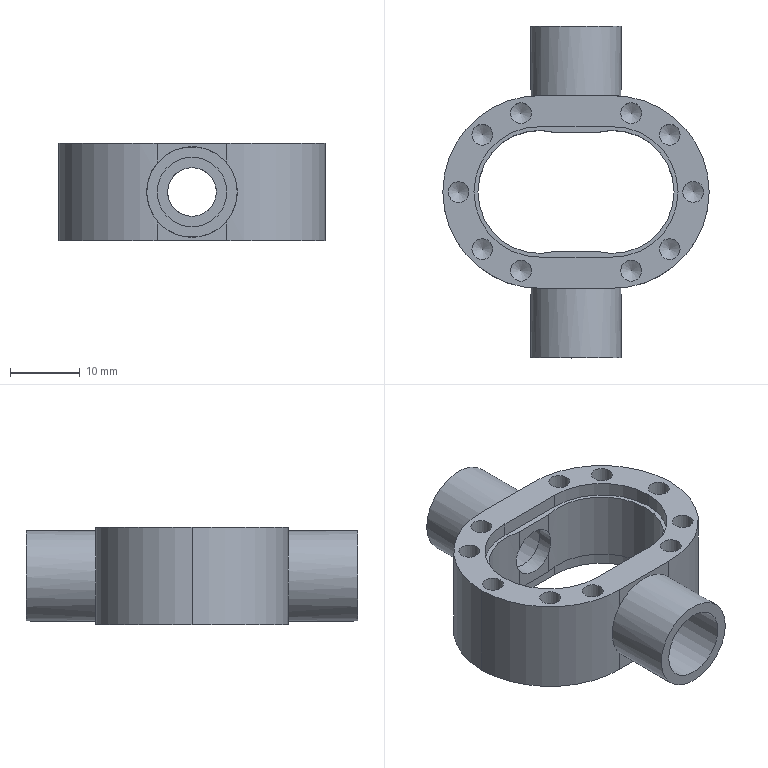Component | NX | CAVITY | 1 solid | 84 faces | volume 6182 mm3 | cylinder 40 | plane 24 | cone 20 | commonest cylinder face diameters 3 x20 18.76 x8 27.68 x4 17.68 x2 13 x2 10 x2 7 x2